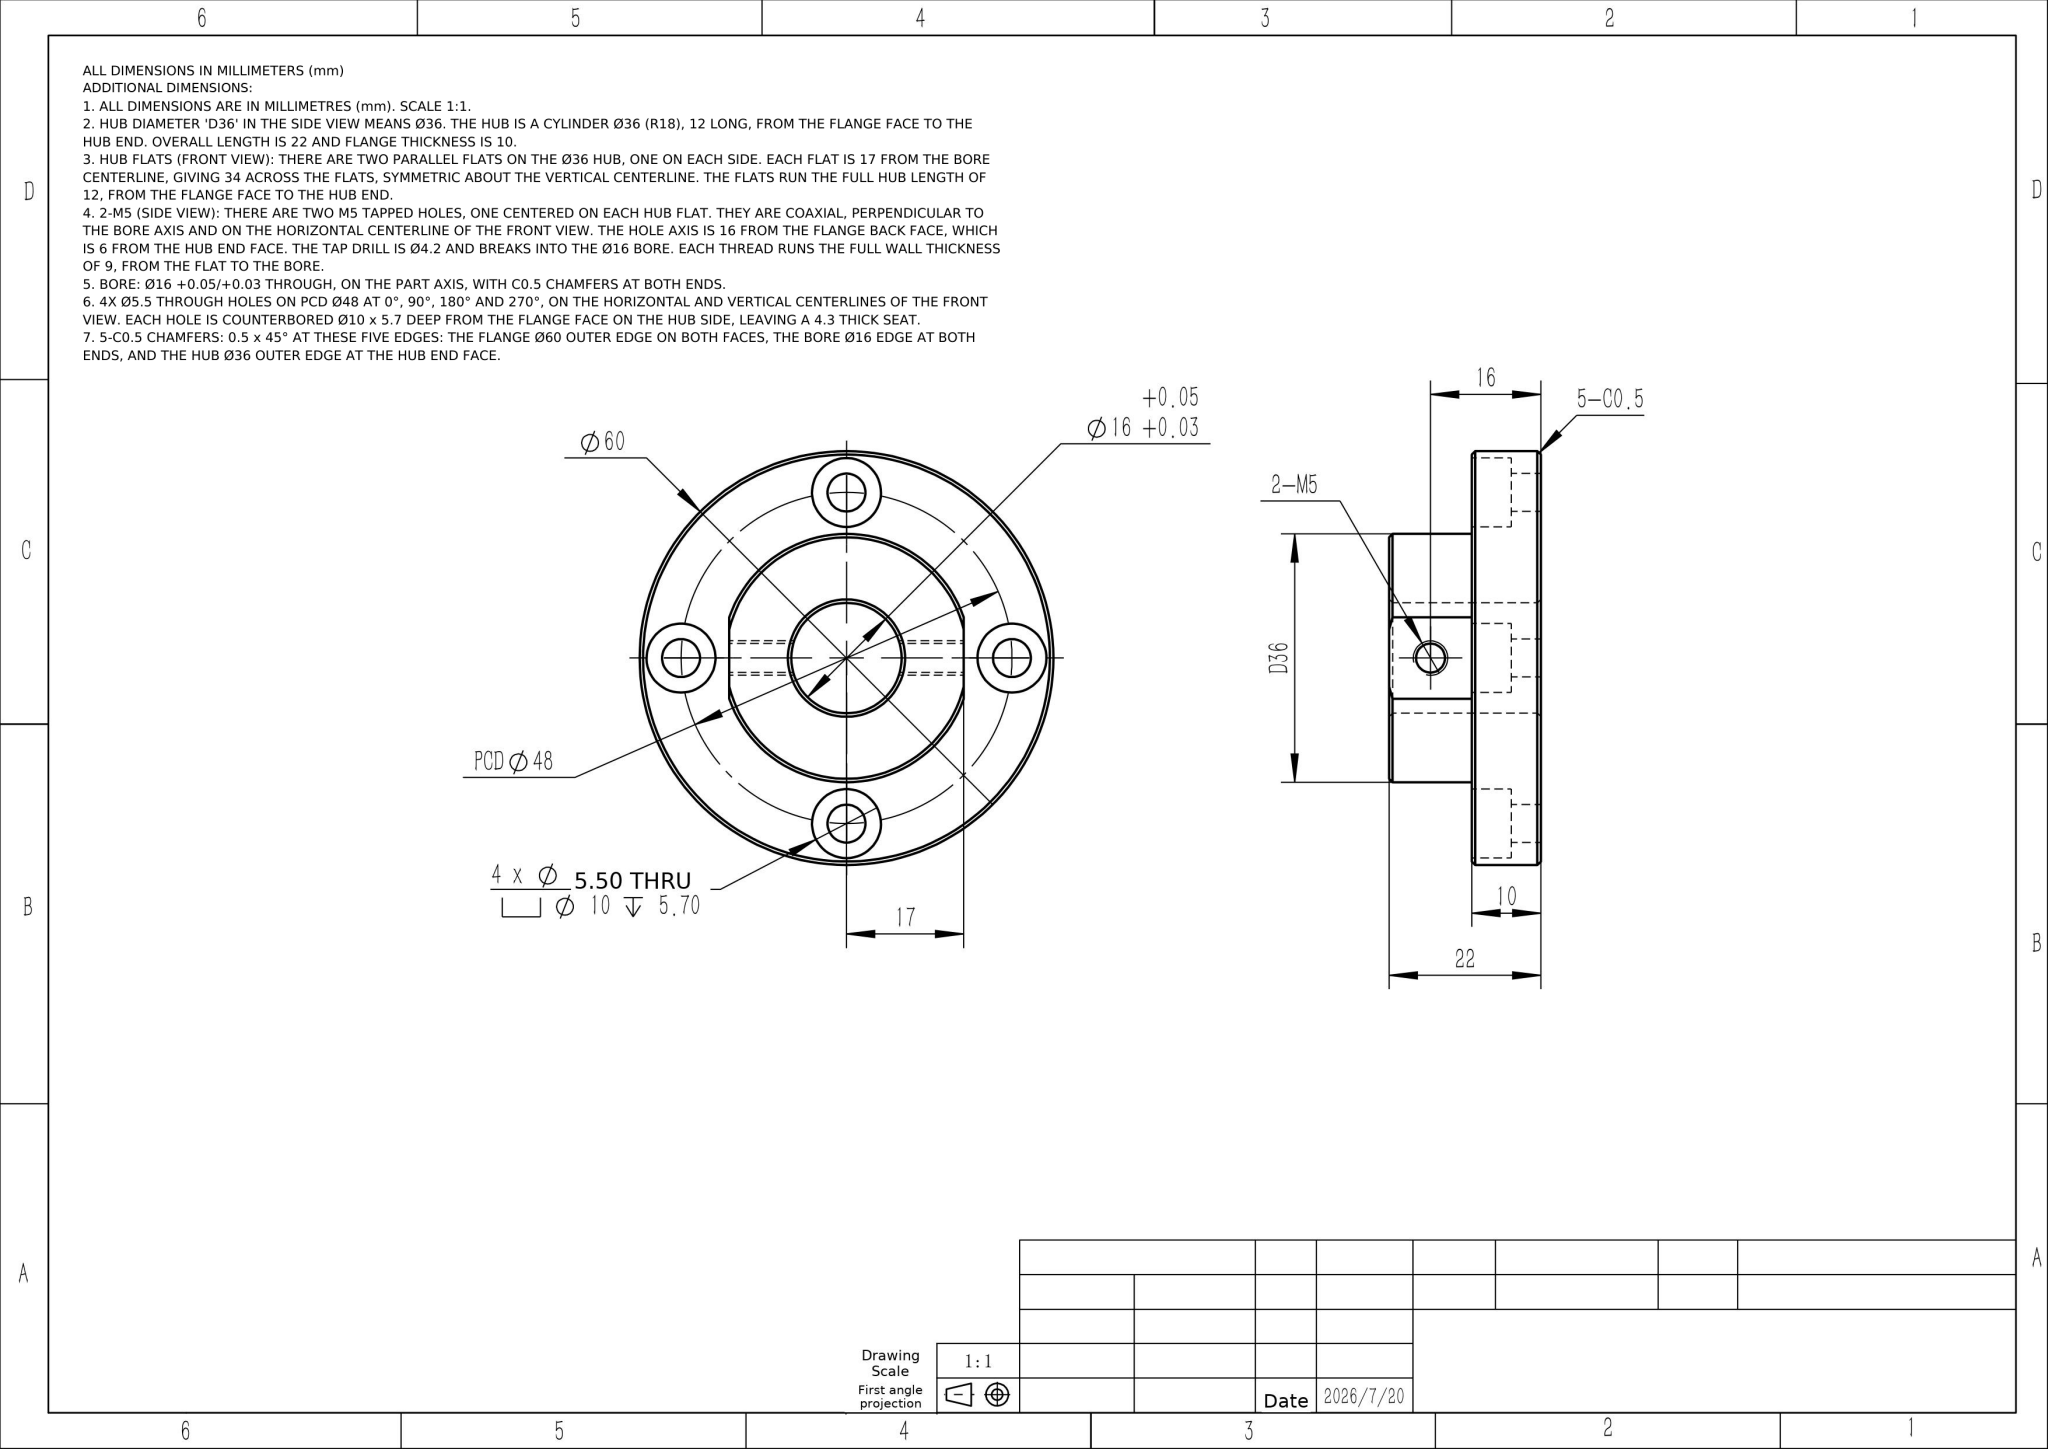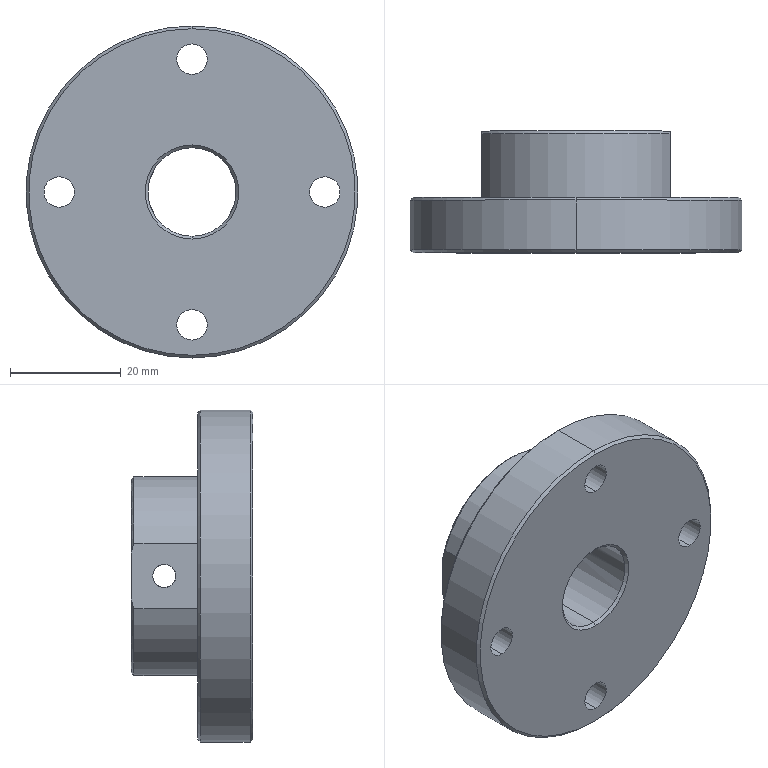Part | NX | mm | Oval Flanged Bore Adapter | 1 solid | 47 faces | box 60 x 22 x 60 mm | volume 33353 mm3 | cylinder 27 | cone 11 | plane 9 | commonest cylinder face diameters 10 x8 5.5 x8 4.2 x4 36 x3 60 x2 16 x2